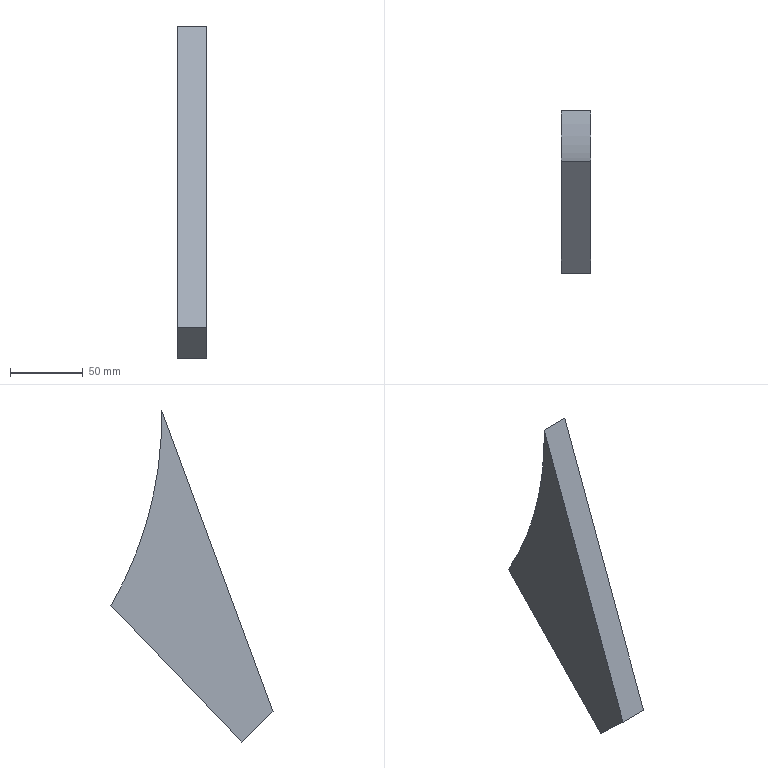Component | SolidWorks | Rebro oslonca izbacivaca-18 | 1 solid | 6 faces | box 20 x 111.57 x 228.63 mm | volume 197199 mm3 | plane 5 | cylinder 1 | commonest cylinder face diameters 521 x1
build123d program:
from build123d import *

# Parameters (mm, degrees)
BOSS_EXTRUDE1_DEPTH = 20


with BuildPart() as part:
    # Sketch1 → Boss-Extrude1 (new body)
    with BuildSketch(Plane.XY):
        with BuildLine():
            Line((161.16, 351.871), (130.25, 225.6))
            ThreePointArc((130.25, 225.6), (185.779, 182.61), (227.807, 126.349))
            Line((227.807, 126.349), (190.3, 344.738))
            Line((190.3, 344.738), (161.16, 351.871))
        make_face()
    extrude(amount=-BOSS_EXTRUDE1_DEPTH)


solid = part.part

# Placed as in the assembly
solid = solid.moved(Location((-710, 0, 0), (-120, 90, 0)))
STEP:
#1=CARTESIAN_POINT('',(-27.953,-13.275,-8.008));
#2=VERTEX_POINT('',#1);
#3=CARTESIAN_POINT('',(-27.953,-12.421,-8.825));
#4=VERTEX_POINT('',#3);
#5=CARTESIAN_POINT('',(-27.953,-12.421,-8.825));
#6=DIRECTION('',(0.,0.7223,-0.6916));
#7=VECTOR('',#6,39.37);
#8=LINE('',#5,#7);
#9=EDGE_CURVE('',#2,#4,#8,.T.);
#10=ORIENTED_EDGE('',*,*,#9,.F.);
#11=CARTESIAN_POINT('',(-28.74,-13.275,-8.008));
#12=VERTEX_POINT('',#11);
#13=CARTESIAN_POINT('',(-28.74,-13.275,-8.008));
#14=DIRECTION('',(1.,0.,0.));
#15=VECTOR('',#14,39.37);
#16=LINE('',#13,#15);
#17=EDGE_CURVE('',#12,#2,#16,.T.);
#18=ORIENTED_EDGE('',*,*,#17,.F.);
#19=CARTESIAN_POINT('',(-28.74,-12.421,-8.825));
#20=VERTEX_POINT('',#19);
#21=CARTESIAN_POINT('',(-28.74,-12.421,-8.825));
#22=DIRECTION('',(0.,0.7223,-0.6916));
#23=VECTOR('',#22,39.37);
#24=LINE('',#21,#23);
#25=EDGE_CURVE('',#12,#20,#24,.T.);
#26=ORIENTED_EDGE('',*,*,#25,.T.);
#27=CARTESIAN_POINT('',(-28.74,-12.421,-8.825));
#28=DIRECTION('',(1.,0.,0.));
#29=VECTOR('',#28,39.37);
#30=LINE('',#27,#29);
#31=EDGE_CURVE('',#20,#4,#30,.T.);
#32=ORIENTED_EDGE('',*,*,#31,.T.);
#33=EDGE_LOOP('',(#10,#18,#26,#32));
#34=FACE_OUTER_BOUND('',#33,.T.);
#35=CARTESIAN_POINT('',(-28.74,-12.421,-8.825));
#36=DIRECTION('',(0.,-0.6916,-0.7223));
#37=DIRECTION('',(0.,0.7223,-0.6916));
#38=AXIS2_PLACEMENT_3D('',#35,#36,#37);
#39=PLANE('',#38);
#40=ADVANCED_FACE('',(#34),#39,.T.);
#41=CARTESIAN_POINT('',(-27.953,-10.254,0.1765));
#42=VERTEX_POINT('',#41);
#43=CARTESIAN_POINT('',(-27.953,-13.275,-8.008));
#44=DIRECTION('',(0.,-0.3462,-0.9382));
#45=VECTOR('',#44,39.37);
#46=LINE('',#43,#45);
#47=EDGE_CURVE('',#42,#2,#46,.T.);
#48=ORIENTED_EDGE('',*,*,#47,.F.);
#49=CARTESIAN_POINT('',(-28.74,-10.254,0.1765));
#50=VERTEX_POINT('',#49);
#51=CARTESIAN_POINT('',(-28.74,-10.254,0.1765));
#52=DIRECTION('',(1.,0.,0.));
#53=VECTOR('',#52,39.37);
#54=LINE('',#51,#53);
#55=EDGE_CURVE('',#50,#42,#54,.T.);
#56=ORIENTED_EDGE('',*,*,#55,.F.);
#57=CARTESIAN_POINT('',(-28.74,-13.275,-8.008));
#58=DIRECTION('',(0.,-0.3462,-0.9382));
#59=VECTOR('',#58,39.37);
#60=LINE('',#57,#59);
#61=EDGE_CURVE('',#50,#12,#60,.T.);
#62=ORIENTED_EDGE('',*,*,#61,.T.);
#63=ORIENTED_EDGE('',*,*,#17,.T.);
#64=EDGE_LOOP('',(#48,#56,#62,#63));
#65=FACE_OUTER_BOUND('',#64,.T.);
#66=CARTESIAN_POINT('',(-28.74,-13.275,-8.008));
#67=DIRECTION('',(0.,-0.9382,0.3462));
#68=DIRECTION('',(0.,-0.3462,-0.9382));
#69=AXIS2_PLACEMENT_3D('',#66,#67,#68);
#70=PLANE('',#69);
#71=ADVANCED_FACE('',(#65),#70,.T.);
#72=CARTESIAN_POINT('',(-27.953,-8.882,-5.128));
#73=VERTEX_POINT('',#72);
#74=CARTESIAN_POINT('',(-27.953,-0.,-0.));
#75=DIRECTION('',(-1.,0.,0.));
#76=DIRECTION('',(0.,-0.866,0.5));
#77=AXIS2_PLACEMENT_3D('',#74,#75,#76);
#78=CIRCLE('',#77,10.256);
#79=EDGE_CURVE('',#73,#42,#78,.T.);
#80=ORIENTED_EDGE('',*,*,#79,.F.);
#81=CARTESIAN_POINT('',(-28.74,-8.882,-5.128));
#82=VERTEX_POINT('',#81);
#83=CARTESIAN_POINT('',(-28.74,-8.882,-5.128));
#84=DIRECTION('',(1.,0.,0.));
#85=VECTOR('',#84,39.37);
#86=LINE('',#83,#85);
#87=EDGE_CURVE('',#82,#73,#86,.T.);
#88=ORIENTED_EDGE('',*,*,#87,.F.);
#89=CARTESIAN_POINT('',(-28.74,-0.,-0.));
#90=DIRECTION('',(-1.,0.,0.));
#91=DIRECTION('',(0.,-0.866,0.5));
#92=AXIS2_PLACEMENT_3D('',#89,#90,#91);
#93=CIRCLE('',#92,10.256);
#94=EDGE_CURVE('',#82,#50,#93,.T.);
#95=ORIENTED_EDGE('',*,*,#94,.T.);
#96=ORIENTED_EDGE('',*,*,#55,.T.);
#97=EDGE_LOOP('',(#80,#88,#95,#96));
#98=FACE_OUTER_BOUND('',#97,.T.);
#99=CARTESIAN_POINT('',(-28.74,-0.,-0.));
#100=DIRECTION('',(1.,0.,0.));
#101=DIRECTION('',(0.,-0.866,0.5));
#102=AXIS2_PLACEMENT_3D('',#99,#100,#101);
#103=CYLINDRICAL_SURFACE('',#102,10.256);
#104=ADVANCED_FACE('',(#98),#103,.F.);
#105=CARTESIAN_POINT('',(-27.953,-12.421,-8.825));
#106=DIRECTION('',(0.,0.6916,0.7223));
#107=VECTOR('',#106,39.37);
#108=LINE('',#105,#107);
#109=EDGE_CURVE('',#4,#73,#108,.T.);
#110=ORIENTED_EDGE('',*,*,#109,.F.);
#111=ORIENTED_EDGE('',*,*,#31,.F.);
#112=CARTESIAN_POINT('',(-28.74,-12.421,-8.825));
#113=DIRECTION('',(0.,0.6916,0.7223));
#114=VECTOR('',#113,39.37);
#115=LINE('',#112,#114);
#116=EDGE_CURVE('',#20,#82,#115,.T.);
#117=ORIENTED_EDGE('',*,*,#116,.T.);
#118=ORIENTED_EDGE('',*,*,#87,.T.);
#119=EDGE_LOOP('',(#110,#111,#117,#118));
#120=FACE_OUTER_BOUND('',#119,.T.);
#121=CARTESIAN_POINT('',(-28.74,-12.421,-8.825));
#122=DIRECTION('',(0.,0.7223,-0.6916));
#123=DIRECTION('',(0.,0.6916,0.7223));
#124=AXIS2_PLACEMENT_3D('',#121,#122,#123);
#125=PLANE('',#124);
#126=ADVANCED_FACE('',(#120),#125,.T.);
#127=ORIENTED_EDGE('',*,*,#25,.F.);
#128=ORIENTED_EDGE('',*,*,#61,.F.);
#129=ORIENTED_EDGE('',*,*,#94,.F.);
#130=ORIENTED_EDGE('',*,*,#116,.F.);
#131=EDGE_LOOP('',(#127,#128,#129,#130));
#132=FACE_OUTER_BOUND('',#131,.T.);
#133=CARTESIAN_POINT('',(-28.74,-0.,-0.));
#134=DIRECTION('',(1.,0.,0.));
#135=DIRECTION('',(0.,-0.866,0.5));
#136=AXIS2_PLACEMENT_3D('',#133,#134,#135);
#137=PLANE('',#136);
#138=ADVANCED_FACE('',(#132),#137,.F.);
#139=ORIENTED_EDGE('',*,*,#9,.T.);
#140=ORIENTED_EDGE('',*,*,#109,.T.);
#141=ORIENTED_EDGE('',*,*,#79,.T.);
#142=ORIENTED_EDGE('',*,*,#47,.T.);
#143=EDGE_LOOP('',(#139,#140,#141,#142));
#144=FACE_OUTER_BOUND('',#143,.T.);
#145=CARTESIAN_POINT('',(-27.953,-0.,-0.));
#146=DIRECTION('',(1.,0.,0.));
#147=DIRECTION('',(0.,-0.866,0.5));
#148=AXIS2_PLACEMENT_3D('',#145,#146,#147);
#149=PLANE('',#148);
#150=ADVANCED_FACE('',(#144),#149,.T.);
#151=CLOSED_SHELL('',(#40,#71,#104,#126,#138,#150));
#152=MANIFOLD_SOLID_BREP('',#151);
#153=CARTESIAN_POINT('',(0.,0.,0.));
#154=DIRECTION('',(0.,0.,1.));
#155=DIRECTION('',(1.,0.,0.));
#156=AXIS2_PLACEMENT_3D('',#153,#154,#155);
#157=(LENGTH_UNIT()NAMED_UNIT(*)SI_UNIT($,.METRE.));
#158=LENGTH_MEASURE_WITH_UNIT(LENGTH_MEASURE(0.0254),#157);
#159=DIMENSIONAL_EXPONENTS(1.,0.,0.,0.,0.,0.,0.);
#160=(CONVERSION_BASED_UNIT('',#158)LENGTH_UNIT()NAMED_UNIT(#159));
#161=UNCERTAINTY_MEASURE_WITH_UNIT(LENGTH_MEASURE(0.00001),#160,'','');
#162=(NAMED_UNIT(*)PLANE_ANGLE_UNIT()SI_UNIT($,.RADIAN.));
#163=(NAMED_UNIT(*)SI_UNIT($,.STERADIAN.)SOLID_ANGLE_UNIT());
#164=(GEOMETRIC_REPRESENTATION_CONTEXT(3)GLOBAL_UNCERTAINTY_ASSIGNED_CONTEXT((#161))GLOBAL_UNIT_ASSIGNED_CONTEXT((#160,#162,#163))REPRESENTATION_CONTEXT('',''));
#165=ADVANCED_BREP_SHAPE_REPRESENTATION('',(#152,#156),#164);
#166=COLOUR_RGB('',0.7922,0.8196,0.9333);
#167=FILL_AREA_STYLE_COLOUR('',#166);
#168=FILL_AREA_STYLE('',(#167));
#169=SURFACE_STYLE_FILL_AREA(#168);
#170=SURFACE_SIDE_STYLE('',(#169));
#171=SURFACE_STYLE_USAGE(.BOTH.,#170);
#172=PRESENTATION_STYLE_ASSIGNMENT((#171));
#173=STYLED_ITEM('',(#172),#152);
#174=(LENGTH_UNIT()NAMED_UNIT(*)SI_UNIT($,.METRE.));
#175=LENGTH_MEASURE_WITH_UNIT(LENGTH_MEASURE(0.0254),#174);
#176=DIMENSIONAL_EXPONENTS(1.,0.,0.,0.,0.,0.,0.);
#177=(CONVERSION_BASED_UNIT('',#175)LENGTH_UNIT()NAMED_UNIT(#176));
#178=UNCERTAINTY_MEASURE_WITH_UNIT(LENGTH_MEASURE(0.00001),#177,'','');
#179=(NAMED_UNIT(*)PLANE_ANGLE_UNIT()SI_UNIT($,.RADIAN.));
#180=(NAMED_UNIT(*)SI_UNIT($,.STERADIAN.)SOLID_ANGLE_UNIT());
#181=(GEOMETRIC_REPRESENTATION_CONTEXT(3)GLOBAL_UNCERTAINTY_ASSIGNED_CONTEXT((#178))GLOBAL_UNIT_ASSIGNED_CONTEXT((#177,#179,#180))REPRESENTATION_CONTEXT('',''));
#182=MECHANICAL_DESIGN_GEOMETRIC_PRESENTATION_REPRESENTATION('',(#173),#181);
#183=PRESENTATION_LAYER_ASSIGNMENT('','',(#173));